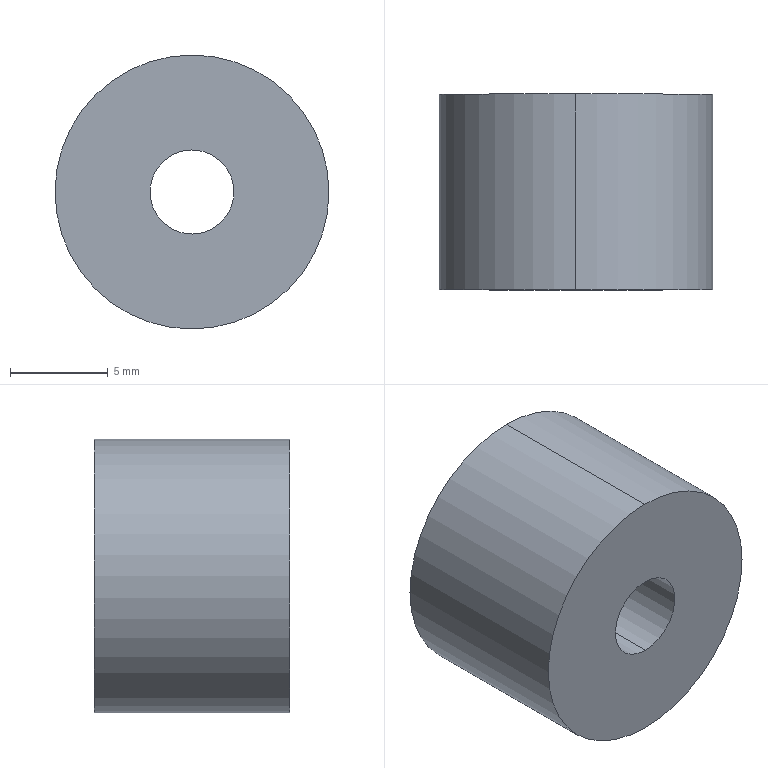Component | SolidWorks | GbgbSpringPostFixingBlockF8-1 | 1 solid | 9 faces | box 14 x 10 x 14 mm | volume 1306 mm3 | cylinder 6 | plane 3 | commonest cylinder face diameters 6.1 x2 14 x2 4.3 x2
build123d program:
from build123d import *

# Parameters (mm, degrees)
SKETCH1_R           = 7
SKETCH1_R_2         = 2.15
BOSS_EXTRUDE1_DEPTH = 5
SKETCH2_R           = 3.05
CUT_EXTRUDE1_DEPTH  = 6


with BuildPart() as part:
    # Sketch1 → Boss-Extrude1 (new, symmetric)
    with BuildSketch(Plane(origin=(0, 0, 0), x_dir=(1, 0, 0), z_dir=(0, 1, 0))):
        with Locations(Location((0, 0, 0), (0, 0, 270))):
            Circle(SKETCH1_R)
        with Locations(Location((0, 0, 0), (0, 0, 270))):
            Circle(SKETCH1_R_2, mode=Mode.SUBTRACT)
    extrude(amount=BOSS_EXTRUDE1_DEPTH, both=True)

    # Sketch2 → Cut-Extrude1 (cut)
    with BuildSketch(Plane.XZ.offset(5)):
        with Locations(Location((0, 0, 0), (0, 0, 270))):
            Circle(SKETCH2_R)
    extrude(amount=-CUT_EXTRUDE1_DEPTH, mode=Mode.SUBTRACT)


solid = part.part

# Placed as in the assembly
solid = solid.moved(Location((55.446, 427.092, 430.232), (180, 0, 0)))
STEP:
#1=COLOUR_RGB('',0.7922,0.8196,0.9333);
#2=FILL_AREA_STYLE_COLOUR('',#1);
#3=FILL_AREA_STYLE('',(#2));
#4=SURFACE_STYLE_FILL_AREA(#3);
#5=SURFACE_SIDE_STYLE('',(#4));
#6=SURFACE_STYLE_USAGE(.BOTH.,#5);
#7=PRESENTATION_STYLE_ASSIGNMENT((#6));
#8=CARTESIAN_POINT('',(2.183,16.775,17.058));
#9=VERTEX_POINT('',#8);
#10=CARTESIAN_POINT('',(2.183,16.775,16.818));
#11=VERTEX_POINT('',#10);
#12=CARTESIAN_POINT('',(2.183,16.775,16.938));
#13=DIRECTION('',(0.,1.,0.));
#14=DIRECTION('',(0.002338,0.,-1.));
#15=AXIS2_PLACEMENT_3D('',#12,#13,#14);
#16=CIRCLE('',#15,0.1201);
#17=EDGE_CURVE('',#9,#11,#16,.T.);
#18=ORIENTED_EDGE('',*,*,#17,.F.);
#19=CARTESIAN_POINT('',(2.183,17.012,17.058));
#20=VERTEX_POINT('',#19);
#21=CARTESIAN_POINT('',(2.183,16.775,17.058));
#22=DIRECTION('',(0.,1.,0.));
#23=VECTOR('',#22,39.37);
#24=LINE('',#21,#23);
#25=EDGE_CURVE('',#9,#20,#24,.T.);
#26=ORIENTED_EDGE('',*,*,#25,.T.);
#27=CARTESIAN_POINT('',(2.183,17.012,16.818));
#28=VERTEX_POINT('',#27);
#29=CARTESIAN_POINT('',(2.183,17.012,16.938));
#30=DIRECTION('',(0.,1.,0.));
#31=DIRECTION('',(0.002338,0.,-1.));
#32=AXIS2_PLACEMENT_3D('',#29,#30,#31);
#33=CIRCLE('',#32,0.1201);
#34=EDGE_CURVE('',#20,#28,#33,.T.);
#35=ORIENTED_EDGE('',*,*,#34,.T.);
#36=CARTESIAN_POINT('',(2.183,16.775,16.818));
#37=DIRECTION('',(0.,1.,0.));
#38=VECTOR('',#37,39.37);
#39=LINE('',#36,#38);
#40=EDGE_CURVE('',#11,#28,#39,.T.);
#41=ORIENTED_EDGE('',*,*,#40,.F.);
#42=EDGE_LOOP('',(#18,#26,#35,#41));
#43=FACE_OUTER_BOUND('',#42,.T.);
#44=CARTESIAN_POINT('',(2.183,16.775,16.938));
#45=DIRECTION('',(0.,1.,0.));
#46=DIRECTION('',(0.002338,0.,-1.));
#47=AXIS2_PLACEMENT_3D('',#44,#45,#46);
#48=CYLINDRICAL_SURFACE('',#47,0.1201);
#49=ADVANCED_FACE('',(#43),#48,.F.);
#50=CARTESIAN_POINT('',(2.182,16.618,17.214));
#51=VERTEX_POINT('',#50);
#52=CARTESIAN_POINT('',(2.184,16.618,16.663));
#53=VERTEX_POINT('',#52);
#54=CARTESIAN_POINT('',(2.183,16.618,16.938));
#55=DIRECTION('',(-0.,-1.,-0.));
#56=DIRECTION('',(-0.002338,0.,1.));
#57=AXIS2_PLACEMENT_3D('',#54,#55,#56);
#58=CIRCLE('',#57,0.2756);
#59=EDGE_CURVE('',#51,#53,#58,.T.);
#60=ORIENTED_EDGE('',*,*,#59,.F.);
#61=CARTESIAN_POINT('',(2.182,17.012,17.214));
#62=VERTEX_POINT('',#61);
#63=CARTESIAN_POINT('',(2.182,16.618,17.214));
#64=DIRECTION('',(0.,1.,0.));
#65=VECTOR('',#64,39.37);
#66=LINE('',#63,#65);
#67=EDGE_CURVE('',#51,#62,#66,.T.);
#68=ORIENTED_EDGE('',*,*,#67,.T.);
#69=CARTESIAN_POINT('',(2.184,17.012,16.663));
#70=VERTEX_POINT('',#69);
#71=CARTESIAN_POINT('',(2.183,17.012,16.938));
#72=DIRECTION('',(-0.,-1.,-0.));
#73=DIRECTION('',(-0.002338,0.,1.));
#74=AXIS2_PLACEMENT_3D('',#71,#72,#73);
#75=CIRCLE('',#74,0.2756);
#76=EDGE_CURVE('',#62,#70,#75,.T.);
#77=ORIENTED_EDGE('',*,*,#76,.T.);
#78=CARTESIAN_POINT('',(2.184,16.618,16.663));
#79=DIRECTION('',(0.,1.,0.));
#80=VECTOR('',#79,39.37);
#81=LINE('',#78,#80);
#82=EDGE_CURVE('',#53,#70,#81,.T.);
#83=ORIENTED_EDGE('',*,*,#82,.F.);
#84=EDGE_LOOP('',(#60,#68,#77,#83));
#85=FACE_OUTER_BOUND('',#84,.T.);
#86=CARTESIAN_POINT('',(2.183,16.618,16.938));
#87=DIRECTION('',(0.,1.,0.));
#88=DIRECTION('',(0.002338,0.,-1.));
#89=AXIS2_PLACEMENT_3D('',#86,#87,#88);
#90=CYLINDRICAL_SURFACE('',#89,0.2756);
#91=ADVANCED_FACE('',(#85),#90,.T.);
#92=CARTESIAN_POINT('',(2.183,16.618,16.854));
#93=VERTEX_POINT('',#92);
#94=CARTESIAN_POINT('',(2.183,16.618,17.023));
#95=VERTEX_POINT('',#94);
#96=CARTESIAN_POINT('',(2.183,16.618,16.938));
#97=DIRECTION('',(-0.,-1.,-0.));
#98=DIRECTION('',(-0.002338,0.,1.));
#99=AXIS2_PLACEMENT_3D('',#96,#97,#98);
#100=CIRCLE('',#99,0.08465);
#101=EDGE_CURVE('',#93,#95,#100,.T.);
#102=ORIENTED_EDGE('',*,*,#101,.T.);
#103=CARTESIAN_POINT('',(2.183,16.775,17.023));
#104=VERTEX_POINT('',#103);
#105=CARTESIAN_POINT('',(2.183,16.618,17.023));
#106=DIRECTION('',(0.,1.,0.));
#107=VECTOR('',#106,39.37);
#108=LINE('',#105,#107);
#109=EDGE_CURVE('',#95,#104,#108,.T.);
#110=ORIENTED_EDGE('',*,*,#109,.T.);
#111=CARTESIAN_POINT('',(2.183,16.775,16.854));
#112=VERTEX_POINT('',#111);
#113=CARTESIAN_POINT('',(2.183,16.775,16.938));
#114=DIRECTION('',(0.,1.,0.));
#115=DIRECTION('',(0.002338,0.,-1.));
#116=AXIS2_PLACEMENT_3D('',#113,#114,#115);
#117=CIRCLE('',#116,0.08465);
#118=EDGE_CURVE('',#104,#112,#117,.T.);
#119=ORIENTED_EDGE('',*,*,#118,.T.);
#120=CARTESIAN_POINT('',(2.183,16.618,16.854));
#121=DIRECTION('',(0.,1.,0.));
#122=VECTOR('',#121,39.37);
#123=LINE('',#120,#122);
#124=EDGE_CURVE('',#93,#112,#123,.T.);
#125=ORIENTED_EDGE('',*,*,#124,.F.);
#126=EDGE_LOOP('',(#102,#110,#119,#125));
#127=FACE_OUTER_BOUND('',#126,.T.);
#128=CARTESIAN_POINT('',(2.183,16.618,16.938));
#129=DIRECTION('',(0.,1.,0.));
#130=DIRECTION('',(0.002338,0.,-1.));
#131=AXIS2_PLACEMENT_3D('',#128,#129,#130);
#132=CYLINDRICAL_SURFACE('',#131,0.08465);
#133=ADVANCED_FACE('',(#127),#132,.F.);
#134=ORIENTED_EDGE('',*,*,#109,.F.);
#135=CARTESIAN_POINT('',(2.183,16.618,16.938));
#136=DIRECTION('',(-0.,-1.,-0.));
#137=DIRECTION('',(-0.002338,0.,1.));
#138=AXIS2_PLACEMENT_3D('',#135,#136,#137);
#139=CIRCLE('',#138,0.08465);
#140=EDGE_CURVE('',#95,#93,#139,.T.);
#141=ORIENTED_EDGE('',*,*,#140,.T.);
#142=ORIENTED_EDGE('',*,*,#124,.T.);
#143=CARTESIAN_POINT('',(2.183,16.775,16.938));
#144=DIRECTION('',(0.,1.,0.));
#145=DIRECTION('',(0.002338,0.,-1.));
#146=AXIS2_PLACEMENT_3D('',#143,#144,#145);
#147=CIRCLE('',#146,0.08465);
#148=EDGE_CURVE('',#112,#104,#147,.T.);
#149=ORIENTED_EDGE('',*,*,#148,.T.);
#150=EDGE_LOOP('',(#134,#141,#142,#149));
#151=FACE_OUTER_BOUND('',#150,.T.);
#152=CARTESIAN_POINT('',(2.183,16.618,16.938));
#153=DIRECTION('',(0.,1.,0.));
#154=DIRECTION('',(0.002338,0.,-1.));
#155=AXIS2_PLACEMENT_3D('',#152,#153,#154);
#156=CYLINDRICAL_SURFACE('',#155,0.08465);
#157=ADVANCED_FACE('',(#151),#156,.F.);
#158=CARTESIAN_POINT('',(2.183,16.618,16.938));
#159=DIRECTION('',(-0.,-1.,-0.));
#160=DIRECTION('',(-0.002338,0.,1.));
#161=AXIS2_PLACEMENT_3D('',#158,#159,#160);
#162=CIRCLE('',#161,0.2756);
#163=EDGE_CURVE('',#53,#51,#162,.T.);
#164=ORIENTED_EDGE('',*,*,#163,.T.);
#165=ORIENTED_EDGE('',*,*,#59,.T.);
#166=EDGE_LOOP('',(#164,#165));
#167=FACE_OUTER_BOUND('',#166,.T.);
#168=ORIENTED_EDGE('',*,*,#101,.F.);
#169=ORIENTED_EDGE('',*,*,#140,.F.);
#170=EDGE_LOOP('',(#168,#169));
#171=FACE_BOUND('',#170,.T.);
#172=CARTESIAN_POINT('',(2.183,16.618,16.938));
#173=DIRECTION('',(-0.,-1.,-0.));
#174=DIRECTION('',(-0.002338,-0.,1.));
#175=AXIS2_PLACEMENT_3D('',#172,#173,#174);
#176=PLANE('',#175);
#177=ADVANCED_FACE('',(#167,#171),#176,.T.);
#178=CARTESIAN_POINT('',(2.183,17.012,16.938));
#179=DIRECTION('',(0.,1.,0.));
#180=DIRECTION('',(0.002338,0.,-1.));
#181=AXIS2_PLACEMENT_3D('',#178,#179,#180);
#182=CIRCLE('',#181,0.1201);
#183=EDGE_CURVE('',#28,#20,#182,.T.);
#184=ORIENTED_EDGE('',*,*,#183,.F.);
#185=ORIENTED_EDGE('',*,*,#34,.F.);
#186=EDGE_LOOP('',(#184,#185));
#187=FACE_BOUND('',#186,.T.);
#188=CARTESIAN_POINT('',(2.183,17.012,16.938));
#189=DIRECTION('',(-0.,-1.,-0.));
#190=DIRECTION('',(-0.002338,0.,1.));
#191=AXIS2_PLACEMENT_3D('',#188,#189,#190);
#192=CIRCLE('',#191,0.2756);
#193=EDGE_CURVE('',#70,#62,#192,.T.);
#194=ORIENTED_EDGE('',*,*,#193,.F.);
#195=ORIENTED_EDGE('',*,*,#76,.F.);
#196=EDGE_LOOP('',(#194,#195));
#197=FACE_OUTER_BOUND('',#196,.T.);
#198=CARTESIAN_POINT('',(2.183,17.012,16.938));
#199=DIRECTION('',(-0.,-1.,-0.));
#200=DIRECTION('',(-0.002338,-0.,1.));
#201=AXIS2_PLACEMENT_3D('',#198,#199,#200);
#202=PLANE('',#201);
#203=ADVANCED_FACE('',(#187,#197),#202,.F.);
#204=ORIENTED_EDGE('',*,*,#67,.F.);
#205=ORIENTED_EDGE('',*,*,#163,.F.);
#206=ORIENTED_EDGE('',*,*,#82,.T.);
#207=ORIENTED_EDGE('',*,*,#193,.T.);
#208=EDGE_LOOP('',(#204,#205,#206,#207));
#209=FACE_OUTER_BOUND('',#208,.T.);
#210=CARTESIAN_POINT('',(2.183,16.618,16.938));
#211=DIRECTION('',(0.,1.,0.));
#212=DIRECTION('',(0.002338,0.,-1.));
#213=AXIS2_PLACEMENT_3D('',#210,#211,#212);
#214=CYLINDRICAL_SURFACE('',#213,0.2756);
#215=ADVANCED_FACE('',(#209),#214,.T.);
#216=ORIENTED_EDGE('',*,*,#25,.F.);
#217=CARTESIAN_POINT('',(2.183,16.775,16.938));
#218=DIRECTION('',(0.,1.,0.));
#219=DIRECTION('',(0.002338,0.,-1.));
#220=AXIS2_PLACEMENT_3D('',#217,#218,#219);
#221=CIRCLE('',#220,0.1201);
#222=EDGE_CURVE('',#11,#9,#221,.T.);
#223=ORIENTED_EDGE('',*,*,#222,.F.);
#224=ORIENTED_EDGE('',*,*,#40,.T.);
#225=ORIENTED_EDGE('',*,*,#183,.T.);
#226=EDGE_LOOP('',(#216,#223,#224,#225));
#227=FACE_OUTER_BOUND('',#226,.T.);
#228=CARTESIAN_POINT('',(2.183,16.775,16.938));
#229=DIRECTION('',(0.,1.,0.));
#230=DIRECTION('',(0.002338,0.,-1.));
#231=AXIS2_PLACEMENT_3D('',#228,#229,#230);
#232=CYLINDRICAL_SURFACE('',#231,0.1201);
#233=ADVANCED_FACE('',(#227),#232,.F.);
#234=ORIENTED_EDGE('',*,*,#148,.F.);
#235=ORIENTED_EDGE('',*,*,#118,.F.);
#236=EDGE_LOOP('',(#234,#235));
#237=FACE_BOUND('',#236,.T.);
#238=ORIENTED_EDGE('',*,*,#222,.T.);
#239=ORIENTED_EDGE('',*,*,#17,.T.);
#240=EDGE_LOOP('',(#238,#239));
#241=FACE_OUTER_BOUND('',#240,.T.);
#242=CARTESIAN_POINT('',(2.183,16.775,16.938));
#243=DIRECTION('',(0.,1.,0.));
#244=DIRECTION('',(0.002338,0.,-1.));
#245=AXIS2_PLACEMENT_3D('',#242,#243,#244);
#246=PLANE('',#245);
#247=ADVANCED_FACE('',(#237,#241),#246,.T.);
#248=CLOSED_SHELL('',(#49,#91,#133,#157,#177,#203,#215,#233,#247));
#249=MANIFOLD_SOLID_BREP('',#248);
#250=STYLED_ITEM('',(#7),#249);
#251=(LENGTH_UNIT()NAMED_UNIT(*)SI_UNIT($,.METRE.));
#252=LENGTH_MEASURE_WITH_UNIT(LENGTH_MEASURE(0.0254),#251);
#253=DIMENSIONAL_EXPONENTS(1.,0.,0.,0.,0.,0.,0.);
#254=(CONVERSION_BASED_UNIT('',#252)LENGTH_UNIT()NAMED_UNIT(#253));
#255=UNCERTAINTY_MEASURE_WITH_UNIT(LENGTH_MEASURE(0.00001),#254,'','');
#256=(NAMED_UNIT(*)PLANE_ANGLE_UNIT()SI_UNIT($,.RADIAN.));
#257=(NAMED_UNIT(*)SI_UNIT($,.STERADIAN.)SOLID_ANGLE_UNIT());
#258=(GEOMETRIC_REPRESENTATION_CONTEXT(3)GLOBAL_UNCERTAINTY_ASSIGNED_CONTEXT((#255))GLOBAL_UNIT_ASSIGNED_CONTEXT((#254,#256,#257))REPRESENTATION_CONTEXT('',''));
#259=MECHANICAL_DESIGN_GEOMETRIC_PRESENTATION_REPRESENTATION('',(#250),#258);
#260=CARTESIAN_POINT('',(0.,0.,0.));
#261=DIRECTION('',(0.,0.,1.));
#262=DIRECTION('',(1.,0.,0.));
#263=AXIS2_PLACEMENT_3D('',#260,#261,#262);
#264=(LENGTH_UNIT()NAMED_UNIT(*)SI_UNIT($,.METRE.));
#265=LENGTH_MEASURE_WITH_UNIT(LENGTH_MEASURE(0.0254),#264);
#266=DIMENSIONAL_EXPONENTS(1.,0.,0.,0.,0.,0.,0.);
#267=(CONVERSION_BASED_UNIT('',#265)LENGTH_UNIT()NAMED_UNIT(#266));
#268=UNCERTAINTY_MEASURE_WITH_UNIT(LENGTH_MEASURE(0.00001),#267,'','');
#269=(NAMED_UNIT(*)PLANE_ANGLE_UNIT()SI_UNIT($,.RADIAN.));
#270=(NAMED_UNIT(*)SI_UNIT($,.STERADIAN.)SOLID_ANGLE_UNIT());
#271=(GEOMETRIC_REPRESENTATION_CONTEXT(3)GLOBAL_UNCERTAINTY_ASSIGNED_CONTEXT((#268))GLOBAL_UNIT_ASSIGNED_CONTEXT((#267,#269,#270))REPRESENTATION_CONTEXT('',''));
#272=ADVANCED_BREP_SHAPE_REPRESENTATION('',(#249,#263),#271);
#273=PRESENTATION_LAYER_ASSIGNMENT('','',(#250));